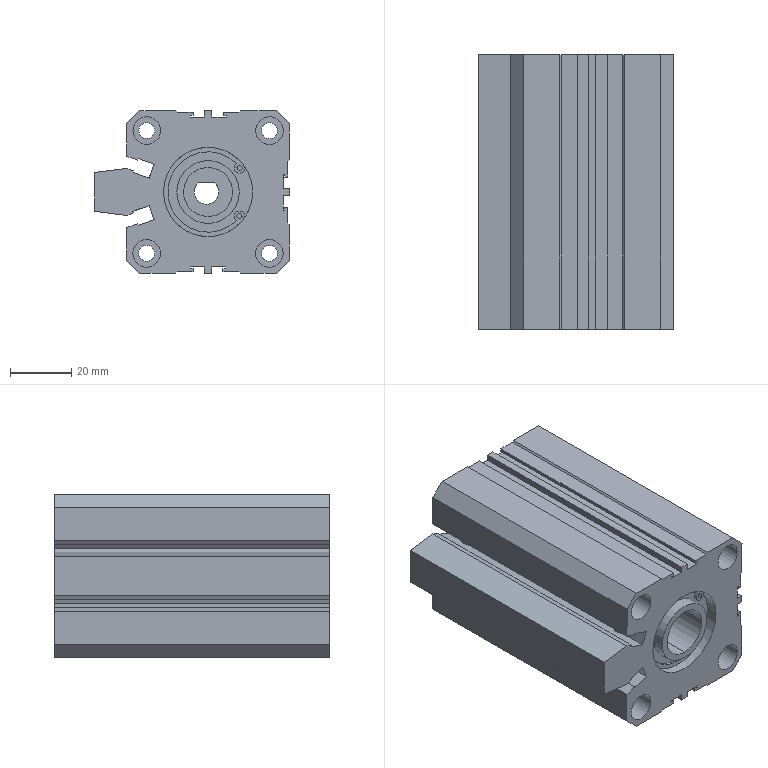Component | SolidWorks | WristClampingAirCTACQS40x50-1_WristClampingCylinderBody-1 | 1 solid | 146 faces | box 63.53 x 89.5 x 53.05 mm | volume 221273 mm3 | plane 97 | cylinder 49 | commonest cylinder face diameters 9 x16 5.2 x8 3.352 x6 1.676 x4 9.728 x4 8 x2 16.5 x2 16 x2